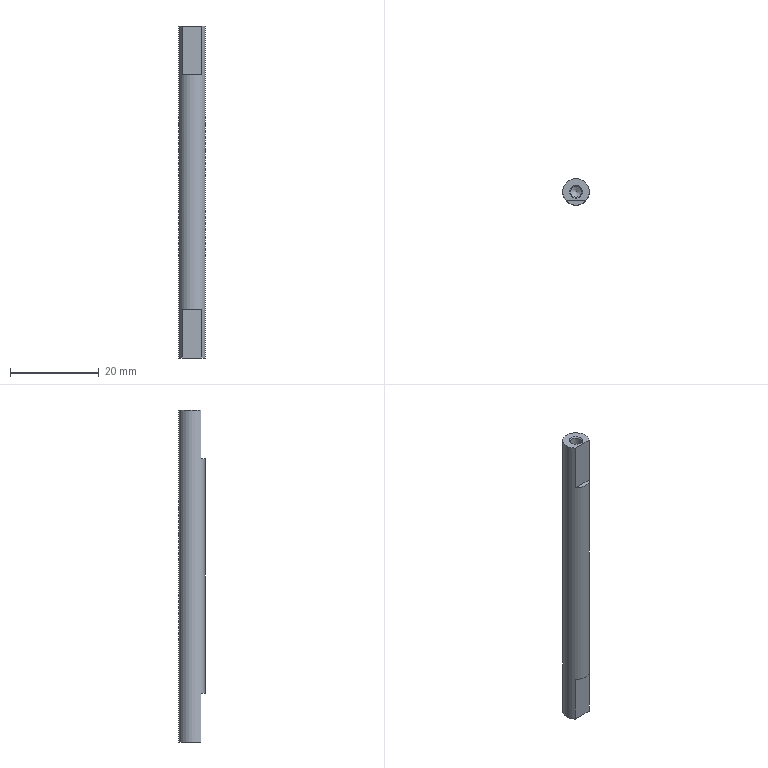Component | NX | DJZ_15_ROTATING_SHAFT_TRAVEL10 | 1 solid | 13 faces | box 6 x 6 x 75 mm | volume 1991 mm3 | plane 6 | cone 4 | cylinder 3 | commonest cylinder face diameters 2.5 x2 6 x1
STEP:
#1=CARTESIAN_POINT('',(0.,0.,0.));
#2=DIRECTION('',(0.,0.,1.));
#3=DIRECTION('',(1.,0.,0.));
#4=AXIS2_PLACEMENT_3D('',#1,#2,#3);
#5=CARTESIAN_POINT('',(1.5,0.,4.5));
#6=VERTEX_POINT('',#5);
#7=CARTESIAN_POINT('',(0.,0.,4.5));
#8=DIRECTION('',(0.,0.,1.));
#9=DIRECTION('',(1.,0.,0.));
#10=AXIS2_PLACEMENT_3D('',#7,#8,#9);
#11=CIRCLE('',#10,1.5);
#12=CARTESIAN_POINT('',(0.,0.,4.5));
#13=DIRECTION('',(0.,0.,1.));
#14=DIRECTION('',(1.,0.,0.));
#15=AXIS2_PLACEMENT_3D('',#12,#13,#14);
#16=PLANE('',#15);
#17=CARTESIAN_POINT('',(0.,0.));
#18=DIRECTION('',(1.,0.));
#19=AXIS2_PLACEMENT_2D('',#17,#18);
#20=CIRCLE('',#19,1.5);
#21=(GEOMETRIC_REPRESENTATION_CONTEXT(2)PARAMETRIC_REPRESENTATION_CONTEXT()REPRESENTATION_CONTEXT('',''));
#22=DEFINITIONAL_REPRESENTATION('',(#20),#21);
#23=PCURVE('',#16,#22);
#24=CARTESIAN_POINT('',(0.,0.,4.5));
#25=DIRECTION('',(0.,0.,-1.));
#26=DIRECTION('',(-1.,0.,0.));
#27=AXIS2_PLACEMENT_3D('',#24,#25,#26);
#28=CONICAL_SURFACE('',#27,1.5,0.7854);
#29=CARTESIAN_POINT('',(9.425,0.));
#30=DIRECTION('',(-1.,0.));
#31=VECTOR('',#30,1.);
#32=LINE('',#29,#31);
#33=(GEOMETRIC_REPRESENTATION_CONTEXT(2)PARAMETRIC_REPRESENTATION_CONTEXT()REPRESENTATION_CONTEXT('',''));
#34=DEFINITIONAL_REPRESENTATION('',(#32),#33);
#35=PCURVE('',#28,#34);
#36=SURFACE_CURVE('',#11,(#23,#35),.PCURVE_S1.);
#37=EDGE_CURVE('',#6,#6,#36,.T.);
#38=ORIENTED_EDGE('',*,*,#37,.T.);
#39=EDGE_LOOP('',(#38));
#40=FACE_BOUND('',#39,.T.);
#41=CARTESIAN_POINT('',(-2.236,-2.,4.5));
#42=VERTEX_POINT('',#41);
#43=CARTESIAN_POINT('',(2.236,-2.,4.5));
#44=VERTEX_POINT('',#43);
#45=CARTESIAN_POINT('',(-2.236,-2.,4.5));
#46=DIRECTION('',(1.,0.,0.));
#47=VECTOR('',#46,1.);
#48=LINE('',#45,#47);
#49=CARTESIAN_POINT('',(-2.236,-2.));
#50=DIRECTION('',(1.,0.));
#51=VECTOR('',#50,1.);
#52=LINE('',#49,#51);
#53=(GEOMETRIC_REPRESENTATION_CONTEXT(2)PARAMETRIC_REPRESENTATION_CONTEXT()REPRESENTATION_CONTEXT('',''));
#54=DEFINITIONAL_REPRESENTATION('',(#52),#53);
#55=PCURVE('',#16,#54);
#56=CARTESIAN_POINT('',(-2.236,-2.,15.5));
#57=DIRECTION('',(0.,1.,0.));
#58=DIRECTION('',(0.,0.,1.));
#59=AXIS2_PLACEMENT_3D('',#56,#57,#58);
#60=PLANE('',#59);
#61=CARTESIAN_POINT('',(-11.,0.));
#62=DIRECTION('',(0.,1.));
#63=VECTOR('',#62,1.);
#64=LINE('',#61,#63);
#65=(GEOMETRIC_REPRESENTATION_CONTEXT(2)PARAMETRIC_REPRESENTATION_CONTEXT()REPRESENTATION_CONTEXT('',''));
#66=DEFINITIONAL_REPRESENTATION('',(#64),#65);
#67=PCURVE('',#60,#66);
#68=SURFACE_CURVE('',#48,(#55,#67),.PCURVE_S1.);
#69=EDGE_CURVE('',#42,#44,#68,.T.);
#70=ORIENTED_EDGE('',*,*,#69,.F.);
#71=CARTESIAN_POINT('',(0.,0.,4.5));
#72=DIRECTION('',(0.,0.,1.));
#73=DIRECTION('',(1.,0.,0.));
#74=AXIS2_PLACEMENT_3D('',#71,#72,#73);
#75=CIRCLE('',#74,3.);
#76=CARTESIAN_POINT('',(0.,0.));
#77=DIRECTION('',(1.,0.));
#78=AXIS2_PLACEMENT_2D('',#76,#77);
#79=CIRCLE('',#78,3.);
#80=(GEOMETRIC_REPRESENTATION_CONTEXT(2)PARAMETRIC_REPRESENTATION_CONTEXT()REPRESENTATION_CONTEXT('',''));
#81=DEFINITIONAL_REPRESENTATION('',(#79),#80);
#82=PCURVE('',#16,#81);
#83=CARTESIAN_POINT('',(0.,0.,79.5));
#84=DIRECTION('',(0.,0.,-1.));
#85=DIRECTION('',(-1.,0.,0.));
#86=AXIS2_PLACEMENT_3D('',#83,#84,#85);
#87=CYLINDRICAL_SURFACE('',#86,3.);
#88=CARTESIAN_POINT('',(15.708,75.));
#89=DIRECTION('',(-1.,0.));
#90=VECTOR('',#89,1.);
#91=LINE('',#88,#90);
#92=(GEOMETRIC_REPRESENTATION_CONTEXT(2)PARAMETRIC_REPRESENTATION_CONTEXT()REPRESENTATION_CONTEXT('',''));
#93=DEFINITIONAL_REPRESENTATION('',(#91),#92);
#94=PCURVE('',#87,#93);
#95=SURFACE_CURVE('',#75,(#82,#94),.PCURVE_S1.);
#96=EDGE_CURVE('',#44,#42,#95,.T.);
#97=ORIENTED_EDGE('',*,*,#96,.F.);
#98=EDGE_LOOP('',(#70,#97));
#99=FACE_BOUND('',#98,.T.);
#100=ADVANCED_FACE('',(#40,#99),#16,.F.);
#101=CARTESIAN_POINT('',(-2.236,-2.,68.5));
#102=VERTEX_POINT('',#101);
#103=CARTESIAN_POINT('',(2.236,-2.,68.5));
#104=VERTEX_POINT('',#103);
#105=CARTESIAN_POINT('',(0.,0.,68.5));
#106=DIRECTION('',(0.,0.,1.));
#107=DIRECTION('',(1.,0.,0.));
#108=AXIS2_PLACEMENT_3D('',#105,#106,#107);
#109=CIRCLE('',#108,3.);
#110=CARTESIAN_POINT('',(15.708,11.));
#111=DIRECTION('',(-1.,0.));
#112=VECTOR('',#111,1.);
#113=LINE('',#110,#112);
#114=(GEOMETRIC_REPRESENTATION_CONTEXT(2)PARAMETRIC_REPRESENTATION_CONTEXT()REPRESENTATION_CONTEXT('',''));
#115=DEFINITIONAL_REPRESENTATION('',(#113),#114);
#116=PCURVE('',#87,#115);
#117=CARTESIAN_POINT('',(0.,0.,68.5));
#118=DIRECTION('',(0.,0.,1.));
#119=DIRECTION('',(1.,0.,0.));
#120=AXIS2_PLACEMENT_3D('',#117,#118,#119);
#121=PLANE('',#120);
#122=CARTESIAN_POINT('',(0.,0.));
#123=DIRECTION('',(1.,0.));
#124=AXIS2_PLACEMENT_2D('',#122,#123);
#125=CIRCLE('',#124,3.);
#126=(GEOMETRIC_REPRESENTATION_CONTEXT(2)PARAMETRIC_REPRESENTATION_CONTEXT()REPRESENTATION_CONTEXT('',''));
#127=DEFINITIONAL_REPRESENTATION('',(#125),#126);
#128=PCURVE('',#121,#127);
#129=SURFACE_CURVE('',#109,(#116,#128),.PCURVE_S1.);
#130=EDGE_CURVE('',#102,#104,#129,.T.);
#131=ORIENTED_EDGE('',*,*,#130,.F.);
#132=CARTESIAN_POINT('',(-2.236,-2.,15.5));
#133=VERTEX_POINT('',#132);
#134=CARTESIAN_POINT('',(-2.236,-2.,68.5));
#135=CARTESIAN_POINT('',(-2.236,-2.,15.5));
#136=B_SPLINE_CURVE_WITH_KNOTS('',1,(#134,#135),.UNSPECIFIED.,.F.,.F.,(2,2),(11.,64.),.PIECEWISE_BEZIER_KNOTS.);
#137=CARTESIAN_POINT('',(11.837,0.));
#138=DIRECTION('',(0.,1.));
#139=VECTOR('',#138,1.);
#140=LINE('',#137,#139);
#141=(GEOMETRIC_REPRESENTATION_CONTEXT(2)PARAMETRIC_REPRESENTATION_CONTEXT()REPRESENTATION_CONTEXT('',''));
#142=DEFINITIONAL_REPRESENTATION('',(#140),#141);
#143=PCURVE('',#87,#142);
#144=CARTESIAN_POINT('',(5.553,0.));
#145=DIRECTION('',(0.,1.));
#146=VECTOR('',#145,1.);
#147=LINE('',#144,#146);
#148=(GEOMETRIC_REPRESENTATION_CONTEXT(2)PARAMETRIC_REPRESENTATION_CONTEXT()REPRESENTATION_CONTEXT('',''));
#149=DEFINITIONAL_REPRESENTATION('',(#147),#148);
#150=PCURVE('',#87,#149);
#151=SEAM_CURVE('',#136,(#143,#150),.PCURVE_S1.);
#152=EDGE_CURVE('',#102,#133,#151,.T.);
#153=ORIENTED_EDGE('',*,*,#152,.T.);
#154=CARTESIAN_POINT('',(2.236,-2.,15.5));
#155=VERTEX_POINT('',#154);
#156=CARTESIAN_POINT('',(0.,0.,15.5));
#157=DIRECTION('',(0.,0.,-1.));
#158=DIRECTION('',(1.,0.,0.));
#159=AXIS2_PLACEMENT_3D('',#156,#157,#158);
#160=CIRCLE('',#159,3.);
#161=CARTESIAN_POINT('',(9.425,64.));
#162=DIRECTION('',(1.,0.));
#163=VECTOR('',#162,1.);
#164=LINE('',#161,#163);
#165=(GEOMETRIC_REPRESENTATION_CONTEXT(2)PARAMETRIC_REPRESENTATION_CONTEXT()REPRESENTATION_CONTEXT('',''));
#166=DEFINITIONAL_REPRESENTATION('',(#164),#165);
#167=PCURVE('',#87,#166);
#168=CARTESIAN_POINT('',(0.,0.,15.5));
#169=DIRECTION('',(0.,0.,-1.));
#170=DIRECTION('',(-1.,0.,0.));
#171=AXIS2_PLACEMENT_3D('',#168,#169,#170);
#172=PLANE('',#171);
#173=CARTESIAN_POINT('',(0.,0.));
#174=DIRECTION('',(-1.,0.));
#175=AXIS2_PLACEMENT_2D('',#173,#174);
#176=CIRCLE('',#175,3.);
#177=(GEOMETRIC_REPRESENTATION_CONTEXT(2)PARAMETRIC_REPRESENTATION_CONTEXT()REPRESENTATION_CONTEXT('',''));
#178=DEFINITIONAL_REPRESENTATION('',(#176),#177);
#179=PCURVE('',#172,#178);
#180=SURFACE_CURVE('',#160,(#167,#179),.PCURVE_S1.);
#181=EDGE_CURVE('',#155,#133,#180,.T.);
#182=ORIENTED_EDGE('',*,*,#181,.F.);
#183=CARTESIAN_POINT('',(2.236,-2.,15.5));
#184=DIRECTION('',(0.,0.,-1.));
#185=VECTOR('',#184,1.);
#186=LINE('',#183,#185);
#187=CARTESIAN_POINT('',(10.155,64.));
#188=DIRECTION('',(0.,1.));
#189=VECTOR('',#188,1.);
#190=LINE('',#187,#189);
#191=(GEOMETRIC_REPRESENTATION_CONTEXT(2)PARAMETRIC_REPRESENTATION_CONTEXT()REPRESENTATION_CONTEXT('',''));
#192=DEFINITIONAL_REPRESENTATION('',(#190),#191);
#193=PCURVE('',#87,#192);
#194=CARTESIAN_POINT('',(0.,4.472));
#195=DIRECTION('',(-1.,0.));
#196=VECTOR('',#195,1.);
#197=LINE('',#194,#196);
#198=(GEOMETRIC_REPRESENTATION_CONTEXT(2)PARAMETRIC_REPRESENTATION_CONTEXT()REPRESENTATION_CONTEXT('',''));
#199=DEFINITIONAL_REPRESENTATION('',(#197),#198);
#200=PCURVE('',#60,#199);
#201=SURFACE_CURVE('',#186,(#193,#200),.PCURVE_S1.);
#202=EDGE_CURVE('',#155,#44,#201,.T.);
#203=ORIENTED_EDGE('',*,*,#202,.T.);
#204=ORIENTED_EDGE('',*,*,#96,.T.);
#205=CARTESIAN_POINT('',(-2.236,-2.,15.5));
#206=DIRECTION('',(0.,0.,1.));
#207=VECTOR('',#206,1.);
#208=LINE('',#205,#207);
#209=CARTESIAN_POINT('',(5.553,64.));
#210=DIRECTION('',(0.,-1.));
#211=VECTOR('',#210,1.);
#212=LINE('',#209,#211);
#213=(GEOMETRIC_REPRESENTATION_CONTEXT(2)PARAMETRIC_REPRESENTATION_CONTEXT()REPRESENTATION_CONTEXT('',''));
#214=DEFINITIONAL_REPRESENTATION('',(#212),#213);
#215=PCURVE('',#87,#214);
#216=CARTESIAN_POINT('',(0.,0.));
#217=DIRECTION('',(1.,0.));
#218=VECTOR('',#217,1.);
#219=LINE('',#216,#218);
#220=(GEOMETRIC_REPRESENTATION_CONTEXT(2)PARAMETRIC_REPRESENTATION_CONTEXT()REPRESENTATION_CONTEXT('',''));
#221=DEFINITIONAL_REPRESENTATION('',(#219),#220);
#222=PCURVE('',#60,#221);
#223=SURFACE_CURVE('',#208,(#215,#222),.PCURVE_S1.);
#224=EDGE_CURVE('',#42,#133,#223,.T.);
#225=ORIENTED_EDGE('',*,*,#224,.T.);
#226=ORIENTED_EDGE('',*,*,#152,.F.);
#227=CARTESIAN_POINT('',(-2.236,-2.,79.5));
#228=VERTEX_POINT('',#227);
#229=CARTESIAN_POINT('',(-2.236,-2.,68.5));
#230=DIRECTION('',(0.,0.,1.));
#231=VECTOR('',#230,1.);
#232=LINE('',#229,#231);
#233=CARTESIAN_POINT('',(5.553,11.));
#234=DIRECTION('',(0.,-1.));
#235=VECTOR('',#234,1.);
#236=LINE('',#233,#235);
#237=(GEOMETRIC_REPRESENTATION_CONTEXT(2)PARAMETRIC_REPRESENTATION_CONTEXT()REPRESENTATION_CONTEXT('',''));
#238=DEFINITIONAL_REPRESENTATION('',(#236),#237);
#239=PCURVE('',#87,#238);
#240=CARTESIAN_POINT('',(2.236,-2.,68.5));
#241=DIRECTION('',(0.,1.,0.));
#242=DIRECTION('',(0.,0.,1.));
#243=AXIS2_PLACEMENT_3D('',#240,#241,#242);
#244=PLANE('',#243);
#245=CARTESIAN_POINT('',(0.,-4.472));
#246=DIRECTION('',(1.,0.));
#247=VECTOR('',#246,1.);
#248=LINE('',#245,#247);
#249=(GEOMETRIC_REPRESENTATION_CONTEXT(2)PARAMETRIC_REPRESENTATION_CONTEXT()REPRESENTATION_CONTEXT('',''));
#250=DEFINITIONAL_REPRESENTATION('',(#248),#249);
#251=PCURVE('',#244,#250);
#252=SURFACE_CURVE('',#232,(#239,#251),.PCURVE_S1.);
#253=EDGE_CURVE('',#102,#228,#252,.T.);
#254=ORIENTED_EDGE('',*,*,#253,.T.);
#255=CARTESIAN_POINT('',(2.236,-2.,79.5));
#256=VERTEX_POINT('',#255);
#257=CARTESIAN_POINT('',(0.,0.,79.5));
#258=DIRECTION('',(0.,0.,1.));
#259=DIRECTION('',(1.,0.,0.));
#260=AXIS2_PLACEMENT_3D('',#257,#258,#259);
#261=CIRCLE('',#260,3.);
#262=CARTESIAN_POINT('',(15.708,0.));
#263=DIRECTION('',(-1.,0.));
#264=VECTOR('',#263,1.);
#265=LINE('',#262,#264);
#266=(GEOMETRIC_REPRESENTATION_CONTEXT(2)PARAMETRIC_REPRESENTATION_CONTEXT()REPRESENTATION_CONTEXT('',''));
#267=DEFINITIONAL_REPRESENTATION('',(#265),#266);
#268=PCURVE('',#87,#267);
#269=CARTESIAN_POINT('',(0.,0.,79.5));
#270=DIRECTION('',(0.,0.,1.));
#271=DIRECTION('',(1.,0.,0.));
#272=AXIS2_PLACEMENT_3D('',#269,#270,#271);
#273=PLANE('',#272);
#274=CARTESIAN_POINT('',(0.,0.));
#275=DIRECTION('',(1.,0.));
#276=AXIS2_PLACEMENT_2D('',#274,#275);
#277=CIRCLE('',#276,3.);
#278=(GEOMETRIC_REPRESENTATION_CONTEXT(2)PARAMETRIC_REPRESENTATION_CONTEXT()REPRESENTATION_CONTEXT('',''));
#279=DEFINITIONAL_REPRESENTATION('',(#277),#278);
#280=PCURVE('',#273,#279);
#281=SURFACE_CURVE('',#261,(#268,#280),.PCURVE_S1.);
#282=EDGE_CURVE('',#256,#228,#281,.T.);
#283=ORIENTED_EDGE('',*,*,#282,.F.);
#284=CARTESIAN_POINT('',(2.236,-2.,68.5));
#285=DIRECTION('',(0.,0.,-1.));
#286=VECTOR('',#285,1.);
#287=LINE('',#284,#286);
#288=CARTESIAN_POINT('',(10.155,11.));
#289=DIRECTION('',(0.,1.));
#290=VECTOR('',#289,1.);
#291=LINE('',#288,#290);
#292=(GEOMETRIC_REPRESENTATION_CONTEXT(2)PARAMETRIC_REPRESENTATION_CONTEXT()REPRESENTATION_CONTEXT('',''));
#293=DEFINITIONAL_REPRESENTATION('',(#291),#292);
#294=PCURVE('',#87,#293);
#295=CARTESIAN_POINT('',(0.,0.));
#296=DIRECTION('',(-1.,0.));
#297=VECTOR('',#296,1.);
#298=LINE('',#295,#297);
#299=(GEOMETRIC_REPRESENTATION_CONTEXT(2)PARAMETRIC_REPRESENTATION_CONTEXT()REPRESENTATION_CONTEXT('',''));
#300=DEFINITIONAL_REPRESENTATION('',(#298),#299);
#301=PCURVE('',#244,#300);
#302=SURFACE_CURVE('',#287,(#294,#301),.PCURVE_S1.);
#303=EDGE_CURVE('',#256,#104,#302,.T.);
#304=ORIENTED_EDGE('',*,*,#303,.T.);
#305=EDGE_LOOP('',(#131,#153,#182,#203,#204,#225,#226,#254,#283,#304));
#306=FACE_BOUND('',#305,.T.);
#307=ADVANCED_FACE('',(#306),#87,.T.);
#308=CARTESIAN_POINT('',(2.236,-2.,79.5));
#309=DIRECTION('',(-1.,0.,0.));
#310=VECTOR('',#309,1.);
#311=LINE('',#308,#310);
#312=CARTESIAN_POINT('',(2.236,-2.));
#313=DIRECTION('',(-1.,0.));
#314=VECTOR('',#313,1.);
#315=LINE('',#312,#314);
#316=(GEOMETRIC_REPRESENTATION_CONTEXT(2)PARAMETRIC_REPRESENTATION_CONTEXT()REPRESENTATION_CONTEXT('',''));
#317=DEFINITIONAL_REPRESENTATION('',(#315),#316);
#318=PCURVE('',#273,#317);
#319=CARTESIAN_POINT('',(11.,0.));
#320=DIRECTION('',(0.,-1.));
#321=VECTOR('',#320,1.);
#322=LINE('',#319,#321);
#323=(GEOMETRIC_REPRESENTATION_CONTEXT(2)PARAMETRIC_REPRESENTATION_CONTEXT()REPRESENTATION_CONTEXT('',''));
#324=DEFINITIONAL_REPRESENTATION('',(#322),#323);
#325=PCURVE('',#244,#324);
#326=SURFACE_CURVE('',#311,(#318,#325),.PCURVE_S1.);
#327=EDGE_CURVE('',#256,#228,#326,.T.);
#328=ORIENTED_EDGE('',*,*,#327,.F.);
#329=ORIENTED_EDGE('',*,*,#282,.T.);
#330=EDGE_LOOP('',(#328,#329));
#331=FACE_BOUND('',#330,.T.);
#332=CARTESIAN_POINT('',(1.5,0.,79.5));
#333=VERTEX_POINT('',#332);
#334=CARTESIAN_POINT('',(0.,0.,79.5));
#335=DIRECTION('',(0.,0.,-1.));
#336=DIRECTION('',(1.,0.,0.));
#337=AXIS2_PLACEMENT_3D('',#334,#335,#336);
#338=CIRCLE('',#337,1.5);
#339=CARTESIAN_POINT('',(1.5,0.));
#340=CARTESIAN_POINT('',(1.5,-2.598));
#341=CARTESIAN_POINT('',(-0.75,-1.299));
#342=CARTESIAN_POINT('',(-3.,-0.));
#343=CARTESIAN_POINT('',(-0.75,1.299));
#344=CARTESIAN_POINT('',(1.5,2.598));
#345=CARTESIAN_POINT('',(1.5,0.));
#346=(BOUNDED_CURVE()B_SPLINE_CURVE(2,(#339,#340,#341,#342,#343,#344,#345),.UNSPECIFIED.,.T.,.F.)B_SPLINE_CURVE_WITH_KNOTS((1,2,2,2,2,1),(-2.094,0.,2.094,4.189,6.283,8.378),.UNSPECIFIED.)CURVE()GEOMETRIC_REPRESENTATION_ITEM()RATIONAL_B_SPLINE_CURVE((1.,0.5,1.,0.5,1.,0.5,1.))REPRESENTATION_ITEM(''));
#347=(GEOMETRIC_REPRESENTATION_CONTEXT(2)PARAMETRIC_REPRESENTATION_CONTEXT()REPRESENTATION_CONTEXT('',''));
#348=DEFINITIONAL_REPRESENTATION('',(#346),#347);
#349=PCURVE('',#273,#348);
#350=CARTESIAN_POINT('',(0.,0.,79.5));
#351=DIRECTION('',(0.,0.,1.));
#352=DIRECTION('',(1.,0.,0.));
#353=AXIS2_PLACEMENT_3D('',#350,#351,#352);
#354=CONICAL_SURFACE('',#353,1.5,0.7854);
#355=CARTESIAN_POINT('',(6.283,0.));
#356=DIRECTION('',(-1.,0.));
#357=VECTOR('',#356,1.);
#358=LINE('',#355,#357);
#359=(GEOMETRIC_REPRESENTATION_CONTEXT(2)PARAMETRIC_REPRESENTATION_CONTEXT()REPRESENTATION_CONTEXT('',''));
#360=DEFINITIONAL_REPRESENTATION('',(#358),#359);
#361=PCURVE('',#354,#360);
#362=SURFACE_CURVE('',#338,(#349,#361),.PCURVE_S1.);
#363=EDGE_CURVE('',#333,#333,#362,.T.);
#364=ORIENTED_EDGE('',*,*,#363,.T.);
#365=EDGE_LOOP('',(#364));
#366=FACE_BOUND('',#365,.T.);
#367=ADVANCED_FACE('',(#331,#366),#273,.T.);
#368=CARTESIAN_POINT('',(-1.25,0.,10.5));
#369=VERTEX_POINT('',#368);
#370=CARTESIAN_POINT('',(1.25,0.,10.5));
#371=VERTEX_POINT('',#370);
#372=CARTESIAN_POINT('',(0.,0.,10.5));
#373=DIRECTION('',(0.,0.,-1.));
#374=DIRECTION('',(1.,0.,0.));
#375=AXIS2_PLACEMENT_3D('',#372,#373,#374);
#376=CIRCLE('',#375,1.25);
#377=CARTESIAN_POINT('',(0.,0.,10.5));
#378=DIRECTION('',(0.,0.,-1.));
#379=DIRECTION('',(-1.,0.,0.));
#380=AXIS2_PLACEMENT_3D('',#377,#378,#379);
#381=CONICAL_SURFACE('',#380,1.25,1.03);
#382=CARTESIAN_POINT('',(-3.142,0.));
#383=DIRECTION('',(1.,0.));
#384=VECTOR('',#383,1.);
#385=LINE('',#382,#384);
#386=(GEOMETRIC_REPRESENTATION_CONTEXT(2)PARAMETRIC_REPRESENTATION_CONTEXT()REPRESENTATION_CONTEXT('',''));
#387=DEFINITIONAL_REPRESENTATION('',(#385),#386);
#388=PCURVE('',#381,#387);
#389=CARTESIAN_POINT('',(0.,0.,4.5));
#390=DIRECTION('',(0.,0.,1.));
#391=DIRECTION('',(1.,0.,0.));
#392=AXIS2_PLACEMENT_3D('',#389,#390,#391);
#393=CYLINDRICAL_SURFACE('',#392,1.25);
#394=CARTESIAN_POINT('',(6.283,6.));
#395=DIRECTION('',(-1.,0.));
#396=VECTOR('',#395,1.);
#397=LINE('',#394,#396);
#398=(GEOMETRIC_REPRESENTATION_CONTEXT(2)PARAMETRIC_REPRESENTATION_CONTEXT()REPRESENTATION_CONTEXT('',''));
#399=DEFINITIONAL_REPRESENTATION('',(#397),#398);
#400=PCURVE('',#393,#399);
#401=SURFACE_CURVE('',#376,(#388,#400),.PCURVE_S1.);
#402=EDGE_CURVE('',#369,#371,#401,.T.);
#403=ORIENTED_EDGE('',*,*,#402,.F.);
#404=CARTESIAN_POINT('',(0.,0.,11.251));
#405=VERTEX_POINT('',#404);
#406=CARTESIAN_POINT('',(0.,-0.,11.251));
#407=CARTESIAN_POINT('',(-1.25,-0.,10.5));
#408=B_SPLINE_CURVE_WITH_KNOTS('',1,(#406,#407),.UNSPECIFIED.,.F.,.F.,(2,2),(-1.458,0.),.PIECEWISE_BEZIER_KNOTS.);
#409=CARTESIAN_POINT('',(0.,0.));
#410=DIRECTION('',(0.,1.));
#411=VECTOR('',#410,1.);
#412=LINE('',#409,#411);
#413=(GEOMETRIC_REPRESENTATION_CONTEXT(2)PARAMETRIC_REPRESENTATION_CONTEXT()REPRESENTATION_CONTEXT('',''));
#414=DEFINITIONAL_REPRESENTATION('',(#412),#413);
#415=PCURVE('',#381,#414);
#416=CARTESIAN_POINT('',(6.283,0.));
#417=DIRECTION('',(0.,1.));
#418=VECTOR('',#417,1.);
#419=LINE('',#416,#418);
#420=(GEOMETRIC_REPRESENTATION_CONTEXT(2)PARAMETRIC_REPRESENTATION_CONTEXT()REPRESENTATION_CONTEXT('',''));
#421=DEFINITIONAL_REPRESENTATION('',(#419),#420);
#422=PCURVE('',#381,#421);
#423=SEAM_CURVE('',#408,(#415,#422),.PCURVE_S1.);
#424=EDGE_CURVE('',#405,#369,#423,.T.);
#425=ORIENTED_EDGE('',*,*,#424,.F.);
#426=ORIENTED_EDGE('',*,*,#424,.T.);
#427=CARTESIAN_POINT('',(0.,0.,10.5));
#428=DIRECTION('',(0.,0.,-1.));
#429=DIRECTION('',(1.,0.,0.));
#430=AXIS2_PLACEMENT_3D('',#427,#428,#429);
#431=CIRCLE('',#430,1.25);
#432=CARTESIAN_POINT('',(3.142,0.));
#433=DIRECTION('',(1.,0.));
#434=VECTOR('',#433,1.);
#435=LINE('',#432,#434);
#436=(GEOMETRIC_REPRESENTATION_CONTEXT(2)PARAMETRIC_REPRESENTATION_CONTEXT()REPRESENTATION_CONTEXT('',''));
#437=DEFINITIONAL_REPRESENTATION('',(#435),#436);
#438=PCURVE('',#381,#437);
#439=CARTESIAN_POINT('',(6.283,6.));
#440=DIRECTION('',(-1.,0.));
#441=VECTOR('',#440,1.);
#442=LINE('',#439,#441);
#443=(GEOMETRIC_REPRESENTATION_CONTEXT(2)PARAMETRIC_REPRESENTATION_CONTEXT()REPRESENTATION_CONTEXT('',''));
#444=DEFINITIONAL_REPRESENTATION('',(#442),#443);
#445=PCURVE('',#393,#444);
#446=SURFACE_CURVE('',#431,(#438,#445),.PCURVE_S1.);
#447=EDGE_CURVE('',#371,#369,#446,.T.);
#448=ORIENTED_EDGE('',*,*,#447,.F.);
#449=EDGE_LOOP('',(#403,#425,#426,#448));
#450=FACE_BOUND('',#449,.F.);
#451=ADVANCED_FACE('',(#450),#381,.F.);
#452=CARTESIAN_POINT('',(1.25,0.,4.75));
#453=VERTEX_POINT('',#452);
#454=CARTESIAN_POINT('',(0.,0.,4.75));
#455=DIRECTION('',(0.,0.,-1.));
#456=DIRECTION('',(1.,0.,0.));
#457=AXIS2_PLACEMENT_3D('',#454,#455,#456);
#458=CIRCLE('',#457,1.25);
#459=CARTESIAN_POINT('',(6.283,0.25));
#460=DIRECTION('',(-1.,0.));
#461=VECTOR('',#460,1.);
#462=LINE('',#459,#461);
#463=(GEOMETRIC_REPRESENTATION_CONTEXT(2)PARAMETRIC_REPRESENTATION_CONTEXT()REPRESENTATION_CONTEXT('',''));
#464=DEFINITIONAL_REPRESENTATION('',(#462),#463);
#465=PCURVE('',#393,#464);
#466=CARTESIAN_POINT('',(3.142,-0.25));
#467=DIRECTION('',(1.,0.));
#468=VECTOR('',#467,1.);
#469=LINE('',#466,#468);
#470=(GEOMETRIC_REPRESENTATION_CONTEXT(2)PARAMETRIC_REPRESENTATION_CONTEXT()REPRESENTATION_CONTEXT('',''));
#471=DEFINITIONAL_REPRESENTATION('',(#469),#470);
#472=PCURVE('',#28,#471);
#473=SURFACE_CURVE('',#458,(#465,#472),.PCURVE_S1.);
#474=EDGE_CURVE('',#453,#453,#473,.T.);
#475=ORIENTED_EDGE('',*,*,#474,.F.);
#476=CARTESIAN_POINT('',(1.25,0.,4.75));
#477=CARTESIAN_POINT('',(1.25,0.,10.5));
#478=B_SPLINE_CURVE_WITH_KNOTS('',1,(#476,#477),.UNSPECIFIED.,.F.,.F.,(2,2),(0.25,6.),.PIECEWISE_BEZIER_KNOTS.);
#479=CARTESIAN_POINT('',(6.283,0.));
#480=DIRECTION('',(0.,1.));
#481=VECTOR('',#480,1.);
#482=LINE('',#479,#481);
#483=(GEOMETRIC_REPRESENTATION_CONTEXT(2)PARAMETRIC_REPRESENTATION_CONTEXT()REPRESENTATION_CONTEXT('',''));
#484=DEFINITIONAL_REPRESENTATION('',(#482),#483);
#485=PCURVE('',#393,#484);
#486=CARTESIAN_POINT('',(0.,0.));
#487=DIRECTION('',(0.,1.));
#488=VECTOR('',#487,1.);
#489=LINE('',#486,#488);
#490=(GEOMETRIC_REPRESENTATION_CONTEXT(2)PARAMETRIC_REPRESENTATION_CONTEXT()REPRESENTATION_CONTEXT('',''));
#491=DEFINITIONAL_REPRESENTATION('',(#489),#490);
#492=PCURVE('',#393,#491);
#493=SEAM_CURVE('',#478,(#485,#492),.PCURVE_S1.);
#494=EDGE_CURVE('',#453,#371,#493,.T.);
#495=ORIENTED_EDGE('',*,*,#494,.T.);
#496=ORIENTED_EDGE('',*,*,#447,.T.);
#497=ORIENTED_EDGE('',*,*,#402,.T.);
#498=ORIENTED_EDGE('',*,*,#494,.F.);
#499=EDGE_LOOP('',(#475,#495,#496,#497,#498));
#500=FACE_BOUND('',#499,.F.);
#501=ADVANCED_FACE('',(#500),#393,.F.);
#502=ORIENTED_EDGE('',*,*,#474,.T.);
#503=CARTESIAN_POINT('',(1.25,0.,4.75));
#504=CARTESIAN_POINT('',(1.5,0.,4.5));
#505=B_SPLINE_CURVE_WITH_KNOTS('',1,(#503,#504),.UNSPECIFIED.,.F.,.F.,(2,2),(-0.3536,0.),.PIECEWISE_BEZIER_KNOTS.);
#506=CARTESIAN_POINT('',(9.425,0.));
#507=DIRECTION('',(0.,1.));
#508=VECTOR('',#507,1.);
#509=LINE('',#506,#508);
#510=(GEOMETRIC_REPRESENTATION_CONTEXT(2)PARAMETRIC_REPRESENTATION_CONTEXT()REPRESENTATION_CONTEXT('',''));
#511=DEFINITIONAL_REPRESENTATION('',(#509),#510);
#512=PCURVE('',#28,#511);
#513=CARTESIAN_POINT('',(3.142,0.));
#514=DIRECTION('',(0.,1.));
#515=VECTOR('',#514,1.);
#516=LINE('',#513,#515);
#517=(GEOMETRIC_REPRESENTATION_CONTEXT(2)PARAMETRIC_REPRESENTATION_CONTEXT()REPRESENTATION_CONTEXT('',''));
#518=DEFINITIONAL_REPRESENTATION('',(#516),#517);
#519=PCURVE('',#28,#518);
#520=SEAM_CURVE('',#505,(#512,#519),.PCURVE_S1.);
#521=EDGE_CURVE('',#453,#6,#520,.T.);
#522=ORIENTED_EDGE('',*,*,#521,.T.);
#523=ORIENTED_EDGE('',*,*,#37,.T.);
#524=ORIENTED_EDGE('',*,*,#521,.F.);
#525=EDGE_LOOP('',(#502,#522,#523,#524));
#526=FACE_BOUND('',#525,.F.);
#527=ADVANCED_FACE('',(#526),#28,.F.);
#528=CARTESIAN_POINT('',(1.25,0.,73.5));
#529=VERTEX_POINT('',#528);
#530=CARTESIAN_POINT('',(-1.25,0.,73.5));
#531=VERTEX_POINT('',#530);
#532=CARTESIAN_POINT('',(0.,0.,73.5));
#533=DIRECTION('',(0.,0.,1.));
#534=DIRECTION('',(-1.,0.,0.));
#535=AXIS2_PLACEMENT_3D('',#532,#533,#534);
#536=CIRCLE('',#535,1.25);
#537=CARTESIAN_POINT('',(0.,0.,73.5));
#538=DIRECTION('',(0.,0.,1.));
#539=DIRECTION('',(1.,0.,0.));
#540=AXIS2_PLACEMENT_3D('',#537,#538,#539);
#541=CONICAL_SURFACE('',#540,1.25,1.03);
#542=CARTESIAN_POINT('',(-3.142,0.));
#543=DIRECTION('',(1.,0.));
#544=VECTOR('',#543,1.);
#545=LINE('',#542,#544);
#546=(GEOMETRIC_REPRESENTATION_CONTEXT(2)PARAMETRIC_REPRESENTATION_CONTEXT()REPRESENTATION_CONTEXT('',''));
#547=DEFINITIONAL_REPRESENTATION('',(#545),#546);
#548=PCURVE('',#541,#547);
#549=CARTESIAN_POINT('',(0.,0.,79.5));
#550=DIRECTION('',(0.,0.,-1.));
#551=DIRECTION('',(-1.,0.,0.));
#552=AXIS2_PLACEMENT_3D('',#549,#550,#551);
#553=CYLINDRICAL_SURFACE('',#552,1.25);
#554=CARTESIAN_POINT('',(12.566,6.));
#555=DIRECTION('',(-1.,0.));
#556=VECTOR('',#555,1.);
#557=LINE('',#554,#556);
#558=(GEOMETRIC_REPRESENTATION_CONTEXT(2)PARAMETRIC_REPRESENTATION_CONTEXT()REPRESENTATION_CONTEXT('',''));
#559=DEFINITIONAL_REPRESENTATION('',(#557),#558);
#560=PCURVE('',#553,#559);
#561=SURFACE_CURVE('',#536,(#548,#560),.PCURVE_S1.);
#562=EDGE_CURVE('',#529,#531,#561,.T.);
#563=ORIENTED_EDGE('',*,*,#562,.F.);
#564=CARTESIAN_POINT('',(0.,0.,72.749));
#565=VERTEX_POINT('',#564);
#566=CARTESIAN_POINT('',(0.,-0.,72.749));
#567=CARTESIAN_POINT('',(1.25,-0.,73.5));
#568=B_SPLINE_CURVE_WITH_KNOTS('',1,(#566,#567),.UNSPECIFIED.,.F.,.F.,(2,2),(-1.458,0.),.PIECEWISE_BEZIER_KNOTS.);
#569=CARTESIAN_POINT('',(0.,0.));
#570=DIRECTION('',(0.,1.));
#571=VECTOR('',#570,1.);
#572=LINE('',#569,#571);
#573=(GEOMETRIC_REPRESENTATION_CONTEXT(2)PARAMETRIC_REPRESENTATION_CONTEXT()REPRESENTATION_CONTEXT('',''));
#574=DEFINITIONAL_REPRESENTATION('',(#572),#573);
#575=PCURVE('',#541,#574);
#576=CARTESIAN_POINT('',(6.283,0.));
#577=DIRECTION('',(0.,1.));
#578=VECTOR('',#577,1.);
#579=LINE('',#576,#578);
#580=(GEOMETRIC_REPRESENTATION_CONTEXT(2)PARAMETRIC_REPRESENTATION_CONTEXT()REPRESENTATION_CONTEXT('',''));
#581=DEFINITIONAL_REPRESENTATION('',(#579),#580);
#582=PCURVE('',#541,#581);
#583=SEAM_CURVE('',#568,(#575,#582),.PCURVE_S1.);
#584=EDGE_CURVE('',#565,#529,#583,.T.);
#585=ORIENTED_EDGE('',*,*,#584,.F.);
#586=ORIENTED_EDGE('',*,*,#584,.T.);
#587=CARTESIAN_POINT('',(0.,0.,73.5));
#588=DIRECTION('',(0.,0.,1.));
#589=DIRECTION('',(-1.,0.,0.));
#590=AXIS2_PLACEMENT_3D('',#587,#588,#589);
#591=CIRCLE('',#590,1.25);
#592=CARTESIAN_POINT('',(3.142,0.));
#593=DIRECTION('',(1.,0.));
#594=VECTOR('',#593,1.);
#595=LINE('',#592,#594);
#596=(GEOMETRIC_REPRESENTATION_CONTEXT(2)PARAMETRIC_REPRESENTATION_CONTEXT()REPRESENTATION_CONTEXT('',''));
#597=DEFINITIONAL_REPRESENTATION('',(#595),#596);
#598=PCURVE('',#541,#597);
#599=CARTESIAN_POINT('',(6.283,6.));
#600=DIRECTION('',(-1.,0.));
#601=VECTOR('',#600,1.);
#602=LINE('',#599,#601);
#603=(GEOMETRIC_REPRESENTATION_CONTEXT(2)PARAMETRIC_REPRESENTATION_CONTEXT()REPRESENTATION_CONTEXT('',''));
#604=DEFINITIONAL_REPRESENTATION('',(#602),#603);
#605=PCURVE('',#553,#604);
#606=SURFACE_CURVE('',#591,(#598,#605),.PCURVE_S1.);
#607=EDGE_CURVE('',#531,#529,#606,.T.);
#608=ORIENTED_EDGE('',*,*,#607,.F.);
#609=EDGE_LOOP('',(#563,#585,#586,#608));
#610=FACE_BOUND('',#609,.F.);
#611=ADVANCED_FACE('',(#610),#541,.F.);
#612=CARTESIAN_POINT('',(1.25,0.,79.25));
#613=VERTEX_POINT('',#612);
#614=CARTESIAN_POINT('',(0.,0.,79.25));
#615=DIRECTION('',(0.,0.,1.));
#616=DIRECTION('',(1.,0.,0.));
#617=AXIS2_PLACEMENT_3D('',#614,#615,#616);
#618=CIRCLE('',#617,1.25);
#619=CARTESIAN_POINT('',(9.425,0.25));
#620=DIRECTION('',(-1.,0.));
#621=VECTOR('',#620,1.);
#622=LINE('',#619,#621);
#623=(GEOMETRIC_REPRESENTATION_CONTEXT(2)PARAMETRIC_REPRESENTATION_CONTEXT()REPRESENTATION_CONTEXT('',''));
#624=DEFINITIONAL_REPRESENTATION('',(#622),#623);
#625=PCURVE('',#553,#624);
#626=CARTESIAN_POINT('',(0.,-0.25));
#627=DIRECTION('',(1.,0.));
#628=VECTOR('',#627,1.);
#629=LINE('',#626,#628);
#630=(GEOMETRIC_REPRESENTATION_CONTEXT(2)PARAMETRIC_REPRESENTATION_CONTEXT()REPRESENTATION_CONTEXT('',''));
#631=DEFINITIONAL_REPRESENTATION('',(#629),#630);
#632=PCURVE('',#354,#631);
#633=SURFACE_CURVE('',#618,(#625,#632),.PCURVE_S1.);
#634=EDGE_CURVE('',#613,#613,#633,.T.);
#635=ORIENTED_EDGE('',*,*,#634,.F.);
#636=CARTESIAN_POINT('',(1.25,0.,79.25));
#637=CARTESIAN_POINT('',(1.25,0.,73.5));
#638=B_SPLINE_CURVE_WITH_KNOTS('',1,(#636,#637),.UNSPECIFIED.,.F.,.F.,(2,2),(0.25,6.),.PIECEWISE_BEZIER_KNOTS.);
#639=CARTESIAN_POINT('',(9.425,0.));
#640=DIRECTION('',(0.,1.));
#641=VECTOR('',#640,1.);
#642=LINE('',#639,#641);
#643=(GEOMETRIC_REPRESENTATION_CONTEXT(2)PARAMETRIC_REPRESENTATION_CONTEXT()REPRESENTATION_CONTEXT('',''));
#644=DEFINITIONAL_REPRESENTATION('',(#642),#643);
#645=PCURVE('',#553,#644);
#646=CARTESIAN_POINT('',(3.142,0.));
#647=DIRECTION('',(0.,1.));
#648=VECTOR('',#647,1.);
#649=LINE('',#646,#648);
#650=(GEOMETRIC_REPRESENTATION_CONTEXT(2)PARAMETRIC_REPRESENTATION_CONTEXT()REPRESENTATION_CONTEXT('',''));
#651=DEFINITIONAL_REPRESENTATION('',(#649),#650);
#652=PCURVE('',#553,#651);
#653=SEAM_CURVE('',#638,(#645,#652),.PCURVE_S1.);
#654=EDGE_CURVE('',#613,#529,#653,.T.);
#655=ORIENTED_EDGE('',*,*,#654,.T.);
#656=ORIENTED_EDGE('',*,*,#562,.T.);
#657=ORIENTED_EDGE('',*,*,#607,.T.);
#658=ORIENTED_EDGE('',*,*,#654,.F.);
#659=EDGE_LOOP('',(#635,#655,#656,#657,#658));
#660=FACE_BOUND('',#659,.F.);
#661=ADVANCED_FACE('',(#660),#553,.F.);
#662=ORIENTED_EDGE('',*,*,#634,.T.);
#663=CARTESIAN_POINT('',(1.25,0.,79.25));
#664=CARTESIAN_POINT('',(1.5,0.,79.5));
#665=B_SPLINE_CURVE_WITH_KNOTS('',1,(#663,#664),.UNSPECIFIED.,.F.,.F.,(2,2),(-0.3536,0.),.PIECEWISE_BEZIER_KNOTS.);
#666=CARTESIAN_POINT('',(6.283,0.));
#667=DIRECTION('',(0.,1.));
#668=VECTOR('',#667,1.);
#669=LINE('',#666,#668);
#670=(GEOMETRIC_REPRESENTATION_CONTEXT(2)PARAMETRIC_REPRESENTATION_CONTEXT()REPRESENTATION_CONTEXT('',''));
#671=DEFINITIONAL_REPRESENTATION('',(#669),#670);
#672=PCURVE('',#354,#671);
#673=CARTESIAN_POINT('',(0.,0.));
#674=DIRECTION('',(0.,1.));
#675=VECTOR('',#674,1.);
#676=LINE('',#673,#675);
#677=(GEOMETRIC_REPRESENTATION_CONTEXT(2)PARAMETRIC_REPRESENTATION_CONTEXT()REPRESENTATION_CONTEXT('',''));
#678=DEFINITIONAL_REPRESENTATION('',(#676),#677);
#679=PCURVE('',#354,#678);
#680=SEAM_CURVE('',#665,(#672,#679),.PCURVE_S1.);
#681=EDGE_CURVE('',#613,#333,#680,.T.);
#682=ORIENTED_EDGE('',*,*,#681,.T.);
#683=ORIENTED_EDGE('',*,*,#363,.T.);
#684=ORIENTED_EDGE('',*,*,#681,.F.);
#685=EDGE_LOOP('',(#662,#682,#683,#684));
#686=FACE_BOUND('',#685,.F.);
#687=ADVANCED_FACE('',(#686),#354,.F.);
#688=ORIENTED_EDGE('',*,*,#69,.T.);
#689=ORIENTED_EDGE('',*,*,#202,.F.);
#690=CARTESIAN_POINT('',(-2.236,-2.,15.5));
#691=DIRECTION('',(-1.,0.,0.));
#692=VECTOR('',#691,1.);
#693=LINE('',#690,#692);
#694=CARTESIAN_POINT('',(0.,0.));
#695=DIRECTION('',(0.,-1.));
#696=VECTOR('',#695,1.);
#697=LINE('',#694,#696);
#698=(GEOMETRIC_REPRESENTATION_CONTEXT(2)PARAMETRIC_REPRESENTATION_CONTEXT()REPRESENTATION_CONTEXT('',''));
#699=DEFINITIONAL_REPRESENTATION('',(#697),#698);
#700=PCURVE('',#60,#699);
#701=CARTESIAN_POINT('',(2.236,-2.));
#702=DIRECTION('',(1.,0.));
#703=VECTOR('',#702,1.);
#704=LINE('',#701,#703);
#705=(GEOMETRIC_REPRESENTATION_CONTEXT(2)PARAMETRIC_REPRESENTATION_CONTEXT()REPRESENTATION_CONTEXT('',''));
#706=DEFINITIONAL_REPRESENTATION('',(#704),#705);
#707=PCURVE('',#172,#706);
#708=SURFACE_CURVE('',#693,(#700,#707),.PCURVE_S1.);
#709=EDGE_CURVE('',#155,#133,#708,.T.);
#710=ORIENTED_EDGE('',*,*,#709,.T.);
#711=ORIENTED_EDGE('',*,*,#224,.F.);
#712=EDGE_LOOP('',(#688,#689,#710,#711));
#713=FACE_BOUND('',#712,.T.);
#714=ADVANCED_FACE('',(#713),#60,.F.);
#715=ORIENTED_EDGE('',*,*,#709,.F.);
#716=ORIENTED_EDGE('',*,*,#181,.T.);
#717=EDGE_LOOP('',(#715,#716));
#718=FACE_BOUND('',#717,.T.);
#719=ADVANCED_FACE('',(#718),#172,.T.);
#720=ORIENTED_EDGE('',*,*,#327,.T.);
#721=ORIENTED_EDGE('',*,*,#253,.F.);
#722=CARTESIAN_POINT('',(2.236,-2.,68.5));
#723=DIRECTION('',(1.,0.,0.));
#724=VECTOR('',#723,1.);
#725=LINE('',#722,#724);
#726=CARTESIAN_POINT('',(0.,0.));
#727=DIRECTION('',(0.,1.));
#728=VECTOR('',#727,1.);
#729=LINE('',#726,#728);
#730=(GEOMETRIC_REPRESENTATION_CONTEXT(2)PARAMETRIC_REPRESENTATION_CONTEXT()REPRESENTATION_CONTEXT('',''));
#731=DEFINITIONAL_REPRESENTATION('',(#729),#730);
#732=PCURVE('',#244,#731);
#733=CARTESIAN_POINT('',(2.236,-2.));
#734=DIRECTION('',(1.,0.));
#735=VECTOR('',#734,1.);
#736=LINE('',#733,#735);
#737=(GEOMETRIC_REPRESENTATION_CONTEXT(2)PARAMETRIC_REPRESENTATION_CONTEXT()REPRESENTATION_CONTEXT('',''));
#738=DEFINITIONAL_REPRESENTATION('',(#736),#737);
#739=PCURVE('',#121,#738);
#740=SURFACE_CURVE('',#725,(#732,#739),.PCURVE_S1.);
#741=EDGE_CURVE('',#102,#104,#740,.T.);
#742=ORIENTED_EDGE('',*,*,#741,.T.);
#743=ORIENTED_EDGE('',*,*,#303,.F.);
#744=EDGE_LOOP('',(#720,#721,#742,#743));
#745=FACE_BOUND('',#744,.T.);
#746=ADVANCED_FACE('',(#745),#244,.F.);
#747=ORIENTED_EDGE('',*,*,#741,.F.);
#748=ORIENTED_EDGE('',*,*,#130,.T.);
#749=EDGE_LOOP('',(#747,#748));
#750=FACE_BOUND('',#749,.T.);
#751=ADVANCED_FACE('',(#750),#121,.T.);
#752=CLOSED_SHELL('',(#100,#307,#367,#451,#501,#527,#611,#661,#687,#714,#719,#746,#751));
#753=MANIFOLD_SOLID_BREP('',#752);
#754=(LENGTH_UNIT()NAMED_UNIT(*)SI_UNIT(.MILLI.,.METRE.));
#755=UNCERTAINTY_MEASURE_WITH_UNIT(LENGTH_MEASURE(0.000005),#754,'','');
#756=(NAMED_UNIT(*)PLANE_ANGLE_UNIT()SI_UNIT($,.RADIAN.));
#757=(NAMED_UNIT(*)SI_UNIT($,.STERADIAN.)SOLID_ANGLE_UNIT());
#758=(GEOMETRIC_REPRESENTATION_CONTEXT(3)GLOBAL_UNCERTAINTY_ASSIGNED_CONTEXT((#755))GLOBAL_UNIT_ASSIGNED_CONTEXT((#754,#756,#757))REPRESENTATION_CONTEXT('',''));
#759=ADVANCED_BREP_SHAPE_REPRESENTATION('',(#4,#753),#758);